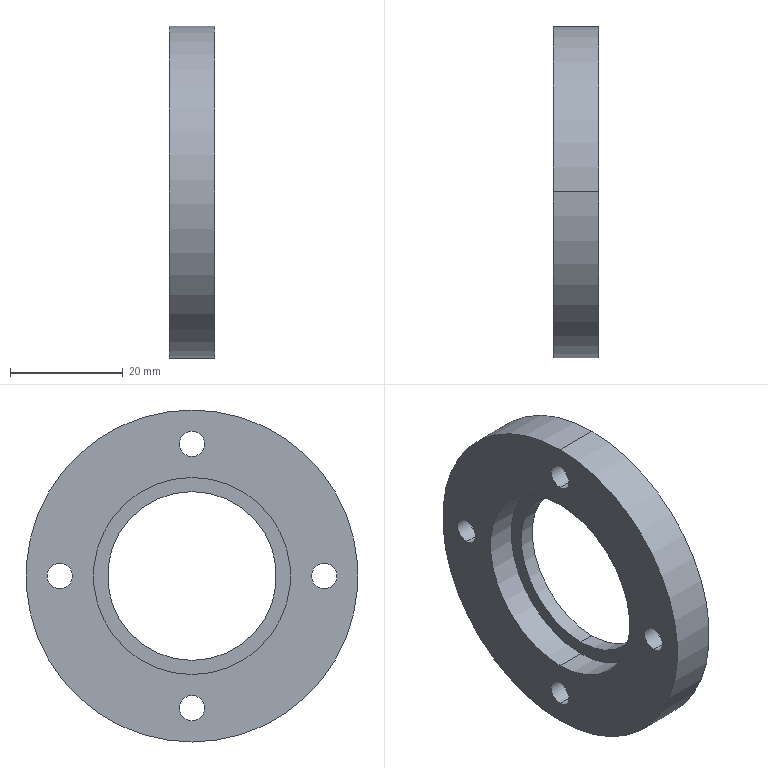Component | SolidWorks | JF21-110.1-33-1-SOLID1-1 | 1 solid | 29 faces | box 8 x 59 x 59 mm | volume 13564 mm3 | cylinder 22 | plane 7 | commonest cylinder face diameters 8.5 x8 4.5 x8 35 x2 59 x2 30 x2
STEP:
#1=COLOUR_RGB('',0.7922,0.8196,0.9333);
#2=FILL_AREA_STYLE_COLOUR('',#1);
#3=FILL_AREA_STYLE('',(#2));
#4=SURFACE_STYLE_FILL_AREA(#3);
#5=SURFACE_SIDE_STYLE('',(#4));
#6=SURFACE_STYLE_USAGE(.BOTH.,#5);
#7=PRESENTATION_STYLE_ASSIGNMENT((#6));
#8=CARTESIAN_POINT('',(17.165,-17.52,23.927));
#9=VERTEX_POINT('',#8);
#10=CARTESIAN_POINT('',(17.165,-17.52,23.593));
#11=VERTEX_POINT('',#10);
#12=CARTESIAN_POINT('',(17.165,-17.52,23.76));
#13=DIRECTION('',(1.,0.,0.));
#14=DIRECTION('',(0.,0.,-1.));
#15=AXIS2_PLACEMENT_3D('',#12,#13,#14);
#16=CIRCLE('',#15,0.1673);
#17=EDGE_CURVE('',#9,#11,#16,.T.);
#18=ORIENTED_EDGE('',*,*,#17,.F.);
#19=CARTESIAN_POINT('',(17.362,-17.52,23.927));
#20=VERTEX_POINT('',#19);
#21=CARTESIAN_POINT('',(17.362,-17.52,23.927));
#22=DIRECTION('',(-1.,0.,0.));
#23=VECTOR('',#22,39.37);
#24=LINE('',#21,#23);
#25=EDGE_CURVE('',#20,#9,#24,.T.);
#26=ORIENTED_EDGE('',*,*,#25,.F.);
#27=CARTESIAN_POINT('',(17.362,-17.52,23.593));
#28=VERTEX_POINT('',#27);
#29=CARTESIAN_POINT('',(17.362,-17.52,23.76));
#30=DIRECTION('',(1.,0.,0.));
#31=DIRECTION('',(0.,0.,-1.));
#32=AXIS2_PLACEMENT_3D('',#29,#30,#31);
#33=CIRCLE('',#32,0.1673);
#34=EDGE_CURVE('',#20,#28,#33,.T.);
#35=ORIENTED_EDGE('',*,*,#34,.T.);
#36=CARTESIAN_POINT('',(17.362,-17.52,23.593));
#37=DIRECTION('',(-1.,0.,0.));
#38=VECTOR('',#37,39.37);
#39=LINE('',#36,#38);
#40=EDGE_CURVE('',#28,#11,#39,.T.);
#41=ORIENTED_EDGE('',*,*,#40,.T.);
#42=EDGE_LOOP('',(#18,#26,#35,#41));
#43=FACE_OUTER_BOUND('',#42,.T.);
#44=CARTESIAN_POINT('',(17.362,-17.52,23.76));
#45=DIRECTION('',(1.,0.,0.));
#46=DIRECTION('',(0.,0.,1.));
#47=AXIS2_PLACEMENT_3D('',#44,#45,#46);
#48=CYLINDRICAL_SURFACE('',#47,0.1673);
#49=ADVANCED_FACE('',(#43),#48,.F.);
#50=CARTESIAN_POINT('',(17.047,-17.52,23.848));
#51=VERTEX_POINT('',#50);
#52=CARTESIAN_POINT('',(17.047,-17.52,23.671));
#53=VERTEX_POINT('',#52);
#54=CARTESIAN_POINT('',(17.047,-17.52,23.76));
#55=DIRECTION('',(1.,0.,0.));
#56=DIRECTION('',(0.,0.,-1.));
#57=AXIS2_PLACEMENT_3D('',#54,#55,#56);
#58=CIRCLE('',#57,0.08858);
#59=EDGE_CURVE('',#51,#53,#58,.T.);
#60=ORIENTED_EDGE('',*,*,#59,.F.);
#61=CARTESIAN_POINT('',(17.165,-17.52,23.848));
#62=VERTEX_POINT('',#61);
#63=CARTESIAN_POINT('',(17.362,-17.52,23.848));
#64=DIRECTION('',(-1.,0.,0.));
#65=VECTOR('',#64,39.37);
#66=LINE('',#63,#65);
#67=EDGE_CURVE('',#62,#51,#66,.T.);
#68=ORIENTED_EDGE('',*,*,#67,.F.);
#69=CARTESIAN_POINT('',(17.165,-17.52,23.671));
#70=VERTEX_POINT('',#69);
#71=CARTESIAN_POINT('',(17.165,-17.52,23.76));
#72=DIRECTION('',(1.,0.,0.));
#73=DIRECTION('',(0.,0.,-1.));
#74=AXIS2_PLACEMENT_3D('',#71,#72,#73);
#75=CIRCLE('',#74,0.08858);
#76=EDGE_CURVE('',#62,#70,#75,.T.);
#77=ORIENTED_EDGE('',*,*,#76,.T.);
#78=CARTESIAN_POINT('',(17.362,-17.52,23.671));
#79=DIRECTION('',(-1.,0.,0.));
#80=VECTOR('',#79,39.37);
#81=LINE('',#78,#80);
#82=EDGE_CURVE('',#70,#53,#81,.T.);
#83=ORIENTED_EDGE('',*,*,#82,.T.);
#84=EDGE_LOOP('',(#60,#68,#77,#83));
#85=FACE_OUTER_BOUND('',#84,.T.);
#86=CARTESIAN_POINT('',(17.362,-17.52,23.76));
#87=DIRECTION('',(1.,0.,0.));
#88=DIRECTION('',(0.,0.,1.));
#89=AXIS2_PLACEMENT_3D('',#86,#87,#88);
#90=CYLINDRICAL_SURFACE('',#89,0.08858);
#91=ADVANCED_FACE('',(#85),#90,.F.);
#92=CARTESIAN_POINT('',(17.165,-18.445,23.002));
#93=VERTEX_POINT('',#92);
#94=CARTESIAN_POINT('',(17.165,-18.445,22.667));
#95=VERTEX_POINT('',#94);
#96=CARTESIAN_POINT('',(17.165,-18.445,22.835));
#97=DIRECTION('',(1.,0.,0.));
#98=DIRECTION('',(0.,0.,-1.));
#99=AXIS2_PLACEMENT_3D('',#96,#97,#98);
#100=CIRCLE('',#99,0.1673);
#101=EDGE_CURVE('',#93,#95,#100,.T.);
#102=ORIENTED_EDGE('',*,*,#101,.F.);
#103=CARTESIAN_POINT('',(17.362,-18.445,23.002));
#104=VERTEX_POINT('',#103);
#105=CARTESIAN_POINT('',(17.362,-18.445,23.002));
#106=DIRECTION('',(-1.,0.,0.));
#107=VECTOR('',#106,39.37);
#108=LINE('',#105,#107);
#109=EDGE_CURVE('',#104,#93,#108,.T.);
#110=ORIENTED_EDGE('',*,*,#109,.F.);
#111=CARTESIAN_POINT('',(17.362,-18.445,22.667));
#112=VERTEX_POINT('',#111);
#113=CARTESIAN_POINT('',(17.362,-18.445,22.835));
#114=DIRECTION('',(1.,0.,0.));
#115=DIRECTION('',(0.,0.,-1.));
#116=AXIS2_PLACEMENT_3D('',#113,#114,#115);
#117=CIRCLE('',#116,0.1673);
#118=EDGE_CURVE('',#104,#112,#117,.T.);
#119=ORIENTED_EDGE('',*,*,#118,.T.);
#120=CARTESIAN_POINT('',(17.362,-18.445,22.667));
#121=DIRECTION('',(-1.,0.,0.));
#122=VECTOR('',#121,39.37);
#123=LINE('',#120,#122);
#124=EDGE_CURVE('',#112,#95,#123,.T.);
#125=ORIENTED_EDGE('',*,*,#124,.T.);
#126=EDGE_LOOP('',(#102,#110,#119,#125));
#127=FACE_OUTER_BOUND('',#126,.T.);
#128=CARTESIAN_POINT('',(17.362,-18.445,22.835));
#129=DIRECTION('',(1.,0.,0.));
#130=DIRECTION('',(0.,0.,1.));
#131=AXIS2_PLACEMENT_3D('',#128,#129,#130);
#132=CYLINDRICAL_SURFACE('',#131,0.1673);
#133=ADVANCED_FACE('',(#127),#132,.F.);
#134=CARTESIAN_POINT('',(17.047,-18.445,22.923));
#135=VERTEX_POINT('',#134);
#136=CARTESIAN_POINT('',(17.047,-18.445,22.746));
#137=VERTEX_POINT('',#136);
#138=CARTESIAN_POINT('',(17.047,-18.445,22.835));
#139=DIRECTION('',(1.,0.,0.));
#140=DIRECTION('',(0.,0.,-1.));
#141=AXIS2_PLACEMENT_3D('',#138,#139,#140);
#142=CIRCLE('',#141,0.08858);
#143=EDGE_CURVE('',#135,#137,#142,.T.);
#144=ORIENTED_EDGE('',*,*,#143,.F.);
#145=CARTESIAN_POINT('',(17.165,-18.445,22.923));
#146=VERTEX_POINT('',#145);
#147=CARTESIAN_POINT('',(17.362,-18.445,22.923));
#148=DIRECTION('',(-1.,0.,0.));
#149=VECTOR('',#148,39.37);
#150=LINE('',#147,#149);
#151=EDGE_CURVE('',#146,#135,#150,.T.);
#152=ORIENTED_EDGE('',*,*,#151,.F.);
#153=CARTESIAN_POINT('',(17.165,-18.445,22.746));
#154=VERTEX_POINT('',#153);
#155=CARTESIAN_POINT('',(17.165,-18.445,22.835));
#156=DIRECTION('',(1.,0.,0.));
#157=DIRECTION('',(0.,0.,-1.));
#158=AXIS2_PLACEMENT_3D('',#155,#156,#157);
#159=CIRCLE('',#158,0.08858);
#160=EDGE_CURVE('',#146,#154,#159,.T.);
#161=ORIENTED_EDGE('',*,*,#160,.T.);
#162=CARTESIAN_POINT('',(17.362,-18.445,22.746));
#163=DIRECTION('',(-1.,0.,0.));
#164=VECTOR('',#163,39.37);
#165=LINE('',#162,#164);
#166=EDGE_CURVE('',#154,#137,#165,.T.);
#167=ORIENTED_EDGE('',*,*,#166,.T.);
#168=EDGE_LOOP('',(#144,#152,#161,#167));
#169=FACE_OUTER_BOUND('',#168,.T.);
#170=CARTESIAN_POINT('',(17.362,-18.445,22.835));
#171=DIRECTION('',(1.,0.,0.));
#172=DIRECTION('',(0.,0.,1.));
#173=AXIS2_PLACEMENT_3D('',#170,#171,#172);
#174=CYLINDRICAL_SURFACE('',#173,0.08858);
#175=ADVANCED_FACE('',(#169),#174,.F.);
#176=CARTESIAN_POINT('',(17.165,-17.52,22.077));
#177=VERTEX_POINT('',#176);
#178=CARTESIAN_POINT('',(17.165,-17.52,21.742));
#179=VERTEX_POINT('',#178);
#180=CARTESIAN_POINT('',(17.165,-17.52,21.909));
#181=DIRECTION('',(1.,0.,0.));
#182=DIRECTION('',(0.,0.,-1.));
#183=AXIS2_PLACEMENT_3D('',#180,#181,#182);
#184=CIRCLE('',#183,0.1673);
#185=EDGE_CURVE('',#177,#179,#184,.T.);
#186=ORIENTED_EDGE('',*,*,#185,.F.);
#187=CARTESIAN_POINT('',(17.362,-17.52,22.077));
#188=VERTEX_POINT('',#187);
#189=CARTESIAN_POINT('',(17.362,-17.52,22.077));
#190=DIRECTION('',(-1.,0.,0.));
#191=VECTOR('',#190,39.37);
#192=LINE('',#189,#191);
#193=EDGE_CURVE('',#188,#177,#192,.T.);
#194=ORIENTED_EDGE('',*,*,#193,.F.);
#195=CARTESIAN_POINT('',(17.362,-17.52,21.742));
#196=VERTEX_POINT('',#195);
#197=CARTESIAN_POINT('',(17.362,-17.52,21.909));
#198=DIRECTION('',(1.,0.,0.));
#199=DIRECTION('',(0.,0.,-1.));
#200=AXIS2_PLACEMENT_3D('',#197,#198,#199);
#201=CIRCLE('',#200,0.1673);
#202=EDGE_CURVE('',#188,#196,#201,.T.);
#203=ORIENTED_EDGE('',*,*,#202,.T.);
#204=CARTESIAN_POINT('',(17.362,-17.52,21.742));
#205=DIRECTION('',(-1.,0.,0.));
#206=VECTOR('',#205,39.37);
#207=LINE('',#204,#206);
#208=EDGE_CURVE('',#196,#179,#207,.T.);
#209=ORIENTED_EDGE('',*,*,#208,.T.);
#210=EDGE_LOOP('',(#186,#194,#203,#209));
#211=FACE_OUTER_BOUND('',#210,.T.);
#212=CARTESIAN_POINT('',(17.362,-17.52,21.909));
#213=DIRECTION('',(1.,0.,0.));
#214=DIRECTION('',(0.,0.,1.));
#215=AXIS2_PLACEMENT_3D('',#212,#213,#214);
#216=CYLINDRICAL_SURFACE('',#215,0.1673);
#217=ADVANCED_FACE('',(#211),#216,.F.);
#218=CARTESIAN_POINT('',(17.047,-17.52,21.998));
#219=VERTEX_POINT('',#218);
#220=CARTESIAN_POINT('',(17.047,-17.52,21.821));
#221=VERTEX_POINT('',#220);
#222=CARTESIAN_POINT('',(17.047,-17.52,21.909));
#223=DIRECTION('',(1.,0.,0.));
#224=DIRECTION('',(0.,0.,-1.));
#225=AXIS2_PLACEMENT_3D('',#222,#223,#224);
#226=CIRCLE('',#225,0.08858);
#227=EDGE_CURVE('',#219,#221,#226,.T.);
#228=ORIENTED_EDGE('',*,*,#227,.F.);
#229=CARTESIAN_POINT('',(17.165,-17.52,21.998));
#230=VERTEX_POINT('',#229);
#231=CARTESIAN_POINT('',(17.362,-17.52,21.998));
#232=DIRECTION('',(-1.,0.,0.));
#233=VECTOR('',#232,39.37);
#234=LINE('',#231,#233);
#235=EDGE_CURVE('',#230,#219,#234,.T.);
#236=ORIENTED_EDGE('',*,*,#235,.F.);
#237=CARTESIAN_POINT('',(17.165,-17.52,21.821));
#238=VERTEX_POINT('',#237);
#239=CARTESIAN_POINT('',(17.165,-17.52,21.909));
#240=DIRECTION('',(1.,0.,0.));
#241=DIRECTION('',(0.,0.,-1.));
#242=AXIS2_PLACEMENT_3D('',#239,#240,#241);
#243=CIRCLE('',#242,0.08858);
#244=EDGE_CURVE('',#230,#238,#243,.T.);
#245=ORIENTED_EDGE('',*,*,#244,.T.);
#246=CARTESIAN_POINT('',(17.362,-17.52,21.821));
#247=DIRECTION('',(-1.,0.,0.));
#248=VECTOR('',#247,39.37);
#249=LINE('',#246,#248);
#250=EDGE_CURVE('',#238,#221,#249,.T.);
#251=ORIENTED_EDGE('',*,*,#250,.T.);
#252=EDGE_LOOP('',(#228,#236,#245,#251));
#253=FACE_OUTER_BOUND('',#252,.T.);
#254=CARTESIAN_POINT('',(17.362,-17.52,21.909));
#255=DIRECTION('',(1.,0.,0.));
#256=DIRECTION('',(0.,0.,1.));
#257=AXIS2_PLACEMENT_3D('',#254,#255,#256);
#258=CYLINDRICAL_SURFACE('',#257,0.08858);
#259=ADVANCED_FACE('',(#253),#258,.F.);
#260=CARTESIAN_POINT('',(17.165,-16.594,23.002));
#261=VERTEX_POINT('',#260);
#262=CARTESIAN_POINT('',(17.165,-16.594,22.667));
#263=VERTEX_POINT('',#262);
#264=CARTESIAN_POINT('',(17.165,-16.594,22.835));
#265=DIRECTION('',(1.,0.,0.));
#266=DIRECTION('',(0.,0.,-1.));
#267=AXIS2_PLACEMENT_3D('',#264,#265,#266);
#268=CIRCLE('',#267,0.1673);
#269=EDGE_CURVE('',#261,#263,#268,.T.);
#270=ORIENTED_EDGE('',*,*,#269,.F.);
#271=CARTESIAN_POINT('',(17.362,-16.594,23.002));
#272=VERTEX_POINT('',#271);
#273=CARTESIAN_POINT('',(17.362,-16.594,23.002));
#274=DIRECTION('',(-1.,0.,0.));
#275=VECTOR('',#274,39.37);
#276=LINE('',#273,#275);
#277=EDGE_CURVE('',#272,#261,#276,.T.);
#278=ORIENTED_EDGE('',*,*,#277,.F.);
#279=CARTESIAN_POINT('',(17.362,-16.594,22.667));
#280=VERTEX_POINT('',#279);
#281=CARTESIAN_POINT('',(17.362,-16.594,22.835));
#282=DIRECTION('',(1.,0.,0.));
#283=DIRECTION('',(0.,0.,-1.));
#284=AXIS2_PLACEMENT_3D('',#281,#282,#283);
#285=CIRCLE('',#284,0.1673);
#286=EDGE_CURVE('',#272,#280,#285,.T.);
#287=ORIENTED_EDGE('',*,*,#286,.T.);
#288=CARTESIAN_POINT('',(17.362,-16.594,22.667));
#289=DIRECTION('',(-1.,0.,0.));
#290=VECTOR('',#289,39.37);
#291=LINE('',#288,#290);
#292=EDGE_CURVE('',#280,#263,#291,.T.);
#293=ORIENTED_EDGE('',*,*,#292,.T.);
#294=EDGE_LOOP('',(#270,#278,#287,#293));
#295=FACE_OUTER_BOUND('',#294,.T.);
#296=CARTESIAN_POINT('',(17.362,-16.594,22.835));
#297=DIRECTION('',(1.,0.,0.));
#298=DIRECTION('',(0.,0.,1.));
#299=AXIS2_PLACEMENT_3D('',#296,#297,#298);
#300=CYLINDRICAL_SURFACE('',#299,0.1673);
#301=ADVANCED_FACE('',(#295),#300,.F.);
#302=CARTESIAN_POINT('',(17.047,-16.594,22.923));
#303=VERTEX_POINT('',#302);
#304=CARTESIAN_POINT('',(17.047,-16.594,22.746));
#305=VERTEX_POINT('',#304);
#306=CARTESIAN_POINT('',(17.047,-16.594,22.835));
#307=DIRECTION('',(1.,0.,0.));
#308=DIRECTION('',(0.,0.,-1.));
#309=AXIS2_PLACEMENT_3D('',#306,#307,#308);
#310=CIRCLE('',#309,0.08858);
#311=EDGE_CURVE('',#303,#305,#310,.T.);
#312=ORIENTED_EDGE('',*,*,#311,.F.);
#313=CARTESIAN_POINT('',(17.165,-16.594,22.923));
#314=VERTEX_POINT('',#313);
#315=CARTESIAN_POINT('',(17.362,-16.594,22.923));
#316=DIRECTION('',(-1.,0.,0.));
#317=VECTOR('',#316,39.37);
#318=LINE('',#315,#317);
#319=EDGE_CURVE('',#314,#303,#318,.T.);
#320=ORIENTED_EDGE('',*,*,#319,.F.);
#321=CARTESIAN_POINT('',(17.165,-16.594,22.746));
#322=VERTEX_POINT('',#321);
#323=CARTESIAN_POINT('',(17.165,-16.594,22.835));
#324=DIRECTION('',(1.,0.,0.));
#325=DIRECTION('',(0.,0.,-1.));
#326=AXIS2_PLACEMENT_3D('',#323,#324,#325);
#327=CIRCLE('',#326,0.08858);
#328=EDGE_CURVE('',#314,#322,#327,.T.);
#329=ORIENTED_EDGE('',*,*,#328,.T.);
#330=CARTESIAN_POINT('',(17.362,-16.594,22.746));
#331=DIRECTION('',(-1.,0.,0.));
#332=VECTOR('',#331,39.37);
#333=LINE('',#330,#332);
#334=EDGE_CURVE('',#322,#305,#333,.T.);
#335=ORIENTED_EDGE('',*,*,#334,.T.);
#336=EDGE_LOOP('',(#312,#320,#329,#335));
#337=FACE_OUTER_BOUND('',#336,.T.);
#338=CARTESIAN_POINT('',(17.362,-16.594,22.835));
#339=DIRECTION('',(1.,0.,0.));
#340=DIRECTION('',(0.,0.,1.));
#341=AXIS2_PLACEMENT_3D('',#338,#339,#340);
#342=CYLINDRICAL_SURFACE('',#341,0.08858);
#343=ADVANCED_FACE('',(#337),#342,.F.);
#344=CARTESIAN_POINT('',(17.252,-17.52,22.146));
#345=VERTEX_POINT('',#344);
#346=CARTESIAN_POINT('',(17.252,-17.52,23.524));
#347=VERTEX_POINT('',#346);
#348=CARTESIAN_POINT('',(17.252,-17.52,22.835));
#349=DIRECTION('',(-1.,0.,0.));
#350=DIRECTION('',(0.,0.,1.));
#351=AXIS2_PLACEMENT_3D('',#348,#349,#350);
#352=CIRCLE('',#351,0.689);
#353=EDGE_CURVE('',#345,#347,#352,.T.);
#354=ORIENTED_EDGE('',*,*,#353,.F.);
#355=CARTESIAN_POINT('',(17.047,-17.52,22.146));
#356=VERTEX_POINT('',#355);
#357=CARTESIAN_POINT('',(17.252,-17.52,22.146));
#358=DIRECTION('',(-1.,0.,0.));
#359=VECTOR('',#358,39.37);
#360=LINE('',#357,#359);
#361=EDGE_CURVE('',#345,#356,#360,.T.);
#362=ORIENTED_EDGE('',*,*,#361,.T.);
#363=CARTESIAN_POINT('',(17.047,-17.52,23.524));
#364=VERTEX_POINT('',#363);
#365=CARTESIAN_POINT('',(17.047,-17.52,22.835));
#366=DIRECTION('',(-1.,0.,0.));
#367=DIRECTION('',(0.,0.,1.));
#368=AXIS2_PLACEMENT_3D('',#365,#366,#367);
#369=CIRCLE('',#368,0.689);
#370=EDGE_CURVE('',#356,#364,#369,.T.);
#371=ORIENTED_EDGE('',*,*,#370,.T.);
#372=CARTESIAN_POINT('',(17.252,-17.52,23.524));
#373=DIRECTION('',(-1.,0.,0.));
#374=VECTOR('',#373,39.37);
#375=LINE('',#372,#374);
#376=EDGE_CURVE('',#347,#364,#375,.T.);
#377=ORIENTED_EDGE('',*,*,#376,.F.);
#378=EDGE_LOOP('',(#354,#362,#371,#377));
#379=FACE_OUTER_BOUND('',#378,.T.);
#380=CARTESIAN_POINT('',(17.252,-17.52,22.835));
#381=DIRECTION('',(-1.,0.,0.));
#382=DIRECTION('',(0.,0.,-1.));
#383=AXIS2_PLACEMENT_3D('',#380,#381,#382);
#384=CYLINDRICAL_SURFACE('',#383,0.689);
#385=ADVANCED_FACE('',(#379),#384,.F.);
#386=CARTESIAN_POINT('',(17.362,-17.52,21.673));
#387=VERTEX_POINT('',#386);
#388=CARTESIAN_POINT('',(17.362,-17.52,23.996));
#389=VERTEX_POINT('',#388);
#390=CARTESIAN_POINT('',(17.362,-17.52,22.835));
#391=DIRECTION('',(1.,0.,0.));
#392=DIRECTION('',(0.,0.,-1.));
#393=AXIS2_PLACEMENT_3D('',#390,#391,#392);
#394=CIRCLE('',#393,1.161);
#395=EDGE_CURVE('',#387,#389,#394,.T.);
#396=ORIENTED_EDGE('',*,*,#395,.F.);
#397=CARTESIAN_POINT('',(17.047,-17.52,21.673));
#398=VERTEX_POINT('',#397);
#399=CARTESIAN_POINT('',(17.362,-17.52,21.673));
#400=DIRECTION('',(-1.,0.,0.));
#401=VECTOR('',#400,39.37);
#402=LINE('',#399,#401);
#403=EDGE_CURVE('',#387,#398,#402,.T.);
#404=ORIENTED_EDGE('',*,*,#403,.T.);
#405=CARTESIAN_POINT('',(17.047,-17.52,23.996));
#406=VERTEX_POINT('',#405);
#407=CARTESIAN_POINT('',(17.047,-17.52,22.835));
#408=DIRECTION('',(1.,0.,0.));
#409=DIRECTION('',(0.,0.,-1.));
#410=AXIS2_PLACEMENT_3D('',#407,#408,#409);
#411=CIRCLE('',#410,1.161);
#412=EDGE_CURVE('',#398,#406,#411,.T.);
#413=ORIENTED_EDGE('',*,*,#412,.T.);
#414=CARTESIAN_POINT('',(17.362,-17.52,23.996));
#415=DIRECTION('',(-1.,0.,0.));
#416=VECTOR('',#415,39.37);
#417=LINE('',#414,#416);
#418=EDGE_CURVE('',#389,#406,#417,.T.);
#419=ORIENTED_EDGE('',*,*,#418,.F.);
#420=EDGE_LOOP('',(#396,#404,#413,#419));
#421=FACE_OUTER_BOUND('',#420,.T.);
#422=CARTESIAN_POINT('',(17.362,-17.52,22.835));
#423=DIRECTION('',(-1.,0.,0.));
#424=DIRECTION('',(0.,0.,-1.));
#425=AXIS2_PLACEMENT_3D('',#422,#423,#424);
#426=CYLINDRICAL_SURFACE('',#425,1.161);
#427=ADVANCED_FACE('',(#421),#426,.T.);
#428=CARTESIAN_POINT('',(17.362,-17.52,22.244));
#429=VERTEX_POINT('',#428);
#430=CARTESIAN_POINT('',(17.362,-17.52,23.425));
#431=VERTEX_POINT('',#430);
#432=CARTESIAN_POINT('',(17.362,-17.52,22.835));
#433=DIRECTION('',(-1.,0.,0.));
#434=DIRECTION('',(0.,0.,1.));
#435=AXIS2_PLACEMENT_3D('',#432,#433,#434);
#436=CIRCLE('',#435,0.5906);
#437=EDGE_CURVE('',#429,#431,#436,.T.);
#438=ORIENTED_EDGE('',*,*,#437,.F.);
#439=CARTESIAN_POINT('',(17.252,-17.52,22.244));
#440=VERTEX_POINT('',#439);
#441=CARTESIAN_POINT('',(17.362,-17.52,22.244));
#442=DIRECTION('',(-1.,0.,0.));
#443=VECTOR('',#442,39.37);
#444=LINE('',#441,#443);
#445=EDGE_CURVE('',#429,#440,#444,.T.);
#446=ORIENTED_EDGE('',*,*,#445,.T.);
#447=CARTESIAN_POINT('',(17.252,-17.52,23.425));
#448=VERTEX_POINT('',#447);
#449=CARTESIAN_POINT('',(17.252,-17.52,22.835));
#450=DIRECTION('',(1.,0.,0.));
#451=DIRECTION('',(0.,0.,1.));
#452=AXIS2_PLACEMENT_3D('',#449,#450,#451);
#453=CIRCLE('',#452,0.5906);
#454=EDGE_CURVE('',#448,#440,#453,.T.);
#455=ORIENTED_EDGE('',*,*,#454,.F.);
#456=CARTESIAN_POINT('',(17.362,-17.52,23.425));
#457=DIRECTION('',(-1.,0.,0.));
#458=VECTOR('',#457,39.37);
#459=LINE('',#456,#458);
#460=EDGE_CURVE('',#431,#448,#459,.T.);
#461=ORIENTED_EDGE('',*,*,#460,.F.);
#462=EDGE_LOOP('',(#438,#446,#455,#461));
#463=FACE_OUTER_BOUND('',#462,.T.);
#464=CARTESIAN_POINT('',(17.362,-17.52,22.835));
#465=DIRECTION('',(-1.,0.,0.));
#466=DIRECTION('',(0.,0.,-1.));
#467=AXIS2_PLACEMENT_3D('',#464,#465,#466);
#468=CYLINDRICAL_SURFACE('',#467,0.5906);
#469=ADVANCED_FACE('',(#463),#468,.F.);
#470=ORIENTED_EDGE('',*,*,#445,.F.);
#471=CARTESIAN_POINT('',(17.362,-17.52,22.835));
#472=DIRECTION('',(-1.,0.,0.));
#473=DIRECTION('',(0.,0.,1.));
#474=AXIS2_PLACEMENT_3D('',#471,#472,#473);
#475=CIRCLE('',#474,0.5906);
#476=EDGE_CURVE('',#431,#429,#475,.T.);
#477=ORIENTED_EDGE('',*,*,#476,.F.);
#478=ORIENTED_EDGE('',*,*,#460,.T.);
#479=CARTESIAN_POINT('',(17.252,-17.52,22.835));
#480=DIRECTION('',(1.,0.,0.));
#481=DIRECTION('',(0.,0.,1.));
#482=AXIS2_PLACEMENT_3D('',#479,#480,#481);
#483=CIRCLE('',#482,0.5906);
#484=EDGE_CURVE('',#440,#448,#483,.T.);
#485=ORIENTED_EDGE('',*,*,#484,.F.);
#486=EDGE_LOOP('',(#470,#477,#478,#485));
#487=FACE_OUTER_BOUND('',#486,.T.);
#488=CARTESIAN_POINT('',(17.362,-17.52,22.835));
#489=DIRECTION('',(-1.,0.,0.));
#490=DIRECTION('',(0.,0.,-1.));
#491=AXIS2_PLACEMENT_3D('',#488,#489,#490);
#492=CYLINDRICAL_SURFACE('',#491,0.5906);
#493=ADVANCED_FACE('',(#487),#492,.F.);
#494=ORIENTED_EDGE('',*,*,#403,.F.);
#495=CARTESIAN_POINT('',(17.362,-17.52,22.835));
#496=DIRECTION('',(1.,0.,0.));
#497=DIRECTION('',(0.,0.,-1.));
#498=AXIS2_PLACEMENT_3D('',#495,#496,#497);
#499=CIRCLE('',#498,1.161);
#500=EDGE_CURVE('',#389,#387,#499,.T.);
#501=ORIENTED_EDGE('',*,*,#500,.F.);
#502=ORIENTED_EDGE('',*,*,#418,.T.);
#503=CARTESIAN_POINT('',(17.047,-17.52,22.835));
#504=DIRECTION('',(1.,0.,0.));
#505=DIRECTION('',(0.,0.,-1.));
#506=AXIS2_PLACEMENT_3D('',#503,#504,#505);
#507=CIRCLE('',#506,1.161);
#508=EDGE_CURVE('',#406,#398,#507,.T.);
#509=ORIENTED_EDGE('',*,*,#508,.T.);
#510=EDGE_LOOP('',(#494,#501,#502,#509));
#511=FACE_OUTER_BOUND('',#510,.T.);
#512=CARTESIAN_POINT('',(17.362,-17.52,22.835));
#513=DIRECTION('',(-1.,0.,0.));
#514=DIRECTION('',(0.,0.,-1.));
#515=AXIS2_PLACEMENT_3D('',#512,#513,#514);
#516=CYLINDRICAL_SURFACE('',#515,1.161);
#517=ADVANCED_FACE('',(#511),#516,.T.);
#518=CARTESIAN_POINT('',(17.362,-17.52,23.76));
#519=DIRECTION('',(1.,0.,0.));
#520=DIRECTION('',(0.,0.,-1.));
#521=AXIS2_PLACEMENT_3D('',#518,#519,#520);
#522=CIRCLE('',#521,0.1673);
#523=EDGE_CURVE('',#28,#20,#522,.T.);
#524=ORIENTED_EDGE('',*,*,#523,.F.);
#525=ORIENTED_EDGE('',*,*,#34,.F.);
#526=EDGE_LOOP('',(#524,#525));
#527=FACE_BOUND('',#526,.T.);
#528=CARTESIAN_POINT('',(17.362,-18.445,22.835));
#529=DIRECTION('',(1.,0.,0.));
#530=DIRECTION('',(0.,0.,-1.));
#531=AXIS2_PLACEMENT_3D('',#528,#529,#530);
#532=CIRCLE('',#531,0.1673);
#533=EDGE_CURVE('',#112,#104,#532,.T.);
#534=ORIENTED_EDGE('',*,*,#533,.F.);
#535=ORIENTED_EDGE('',*,*,#118,.F.);
#536=EDGE_LOOP('',(#534,#535));
#537=FACE_BOUND('',#536,.T.);
#538=CARTESIAN_POINT('',(17.362,-17.52,21.909));
#539=DIRECTION('',(1.,0.,0.));
#540=DIRECTION('',(0.,0.,-1.));
#541=AXIS2_PLACEMENT_3D('',#538,#539,#540);
#542=CIRCLE('',#541,0.1673);
#543=EDGE_CURVE('',#196,#188,#542,.T.);
#544=ORIENTED_EDGE('',*,*,#543,.F.);
#545=ORIENTED_EDGE('',*,*,#202,.F.);
#546=EDGE_LOOP('',(#544,#545));
#547=FACE_BOUND('',#546,.T.);
#548=CARTESIAN_POINT('',(17.362,-16.594,22.835));
#549=DIRECTION('',(1.,0.,0.));
#550=DIRECTION('',(0.,0.,-1.));
#551=AXIS2_PLACEMENT_3D('',#548,#549,#550);
#552=CIRCLE('',#551,0.1673);
#553=EDGE_CURVE('',#280,#272,#552,.T.);
#554=ORIENTED_EDGE('',*,*,#553,.F.);
#555=ORIENTED_EDGE('',*,*,#286,.F.);
#556=EDGE_LOOP('',(#554,#555));
#557=FACE_BOUND('',#556,.T.);
#558=ORIENTED_EDGE('',*,*,#476,.T.);
#559=ORIENTED_EDGE('',*,*,#437,.T.);
#560=EDGE_LOOP('',(#558,#559));
#561=FACE_BOUND('',#560,.T.);
#562=ORIENTED_EDGE('',*,*,#500,.T.);
#563=ORIENTED_EDGE('',*,*,#395,.T.);
#564=EDGE_LOOP('',(#562,#563));
#565=FACE_OUTER_BOUND('',#564,.T.);
#566=CARTESIAN_POINT('',(17.362,-17.52,22.835));
#567=DIRECTION('',(1.,0.,0.));
#568=DIRECTION('',(0.,0.,1.));
#569=AXIS2_PLACEMENT_3D('',#566,#567,#568);
#570=PLANE('',#569);
#571=ADVANCED_FACE('',(#527,#537,#547,#557,#561,#565),#570,.T.);
#572=CARTESIAN_POINT('',(17.047,-17.52,23.76));
#573=DIRECTION('',(1.,0.,0.));
#574=DIRECTION('',(0.,0.,-1.));
#575=AXIS2_PLACEMENT_3D('',#572,#573,#574);
#576=CIRCLE('',#575,0.08858);
#577=EDGE_CURVE('',#53,#51,#576,.T.);
#578=ORIENTED_EDGE('',*,*,#577,.T.);
#579=ORIENTED_EDGE('',*,*,#59,.T.);
#580=EDGE_LOOP('',(#578,#579));
#581=FACE_BOUND('',#580,.T.);
#582=CARTESIAN_POINT('',(17.047,-18.445,22.835));
#583=DIRECTION('',(1.,0.,0.));
#584=DIRECTION('',(0.,0.,-1.));
#585=AXIS2_PLACEMENT_3D('',#582,#583,#584);
#586=CIRCLE('',#585,0.08858);
#587=EDGE_CURVE('',#137,#135,#586,.T.);
#588=ORIENTED_EDGE('',*,*,#587,.T.);
#589=ORIENTED_EDGE('',*,*,#143,.T.);
#590=EDGE_LOOP('',(#588,#589));
#591=FACE_BOUND('',#590,.T.);
#592=CARTESIAN_POINT('',(17.047,-17.52,21.909));
#593=DIRECTION('',(1.,0.,0.));
#594=DIRECTION('',(0.,0.,-1.));
#595=AXIS2_PLACEMENT_3D('',#592,#593,#594);
#596=CIRCLE('',#595,0.08858);
#597=EDGE_CURVE('',#221,#219,#596,.T.);
#598=ORIENTED_EDGE('',*,*,#597,.T.);
#599=ORIENTED_EDGE('',*,*,#227,.T.);
#600=EDGE_LOOP('',(#598,#599));
#601=FACE_BOUND('',#600,.T.);
#602=CARTESIAN_POINT('',(17.047,-16.594,22.835));
#603=DIRECTION('',(1.,0.,0.));
#604=DIRECTION('',(0.,0.,-1.));
#605=AXIS2_PLACEMENT_3D('',#602,#603,#604);
#606=CIRCLE('',#605,0.08858);
#607=EDGE_CURVE('',#305,#303,#606,.T.);
#608=ORIENTED_EDGE('',*,*,#607,.T.);
#609=ORIENTED_EDGE('',*,*,#311,.T.);
#610=EDGE_LOOP('',(#608,#609));
#611=FACE_BOUND('',#610,.T.);
#612=CARTESIAN_POINT('',(17.047,-17.52,22.835));
#613=DIRECTION('',(-1.,0.,0.));
#614=DIRECTION('',(0.,0.,1.));
#615=AXIS2_PLACEMENT_3D('',#612,#613,#614);
#616=CIRCLE('',#615,0.689);
#617=EDGE_CURVE('',#364,#356,#616,.T.);
#618=ORIENTED_EDGE('',*,*,#617,.F.);
#619=ORIENTED_EDGE('',*,*,#370,.F.);
#620=EDGE_LOOP('',(#618,#619));
#621=FACE_BOUND('',#620,.T.);
#622=ORIENTED_EDGE('',*,*,#508,.F.);
#623=ORIENTED_EDGE('',*,*,#412,.F.);
#624=EDGE_LOOP('',(#622,#623));
#625=FACE_OUTER_BOUND('',#624,.T.);
#626=CARTESIAN_POINT('',(17.047,-17.52,22.835));
#627=DIRECTION('',(1.,0.,0.));
#628=DIRECTION('',(0.,0.,1.));
#629=AXIS2_PLACEMENT_3D('',#626,#627,#628);
#630=PLANE('',#629);
#631=ADVANCED_FACE('',(#581,#591,#601,#611,#621,#625),#630,.F.);
#632=CARTESIAN_POINT('',(17.252,-17.52,22.835));
#633=DIRECTION('',(-1.,0.,0.));
#634=DIRECTION('',(0.,0.,1.));
#635=AXIS2_PLACEMENT_3D('',#632,#633,#634);
#636=CIRCLE('',#635,0.689);
#637=EDGE_CURVE('',#347,#345,#636,.T.);
#638=ORIENTED_EDGE('',*,*,#637,.T.);
#639=ORIENTED_EDGE('',*,*,#353,.T.);
#640=EDGE_LOOP('',(#638,#639));
#641=FACE_OUTER_BOUND('',#640,.T.);
#642=ORIENTED_EDGE('',*,*,#454,.T.);
#643=ORIENTED_EDGE('',*,*,#484,.T.);
#644=EDGE_LOOP('',(#642,#643));
#645=FACE_BOUND('',#644,.T.);
#646=CARTESIAN_POINT('',(17.252,-17.52,22.835));
#647=DIRECTION('',(-1.,0.,0.));
#648=DIRECTION('',(0.,0.,-1.));
#649=AXIS2_PLACEMENT_3D('',#646,#647,#648);
#650=PLANE('',#649);
#651=ADVANCED_FACE('',(#641,#645),#650,.T.);
#652=ORIENTED_EDGE('',*,*,#361,.F.);
#653=ORIENTED_EDGE('',*,*,#637,.F.);
#654=ORIENTED_EDGE('',*,*,#376,.T.);
#655=ORIENTED_EDGE('',*,*,#617,.T.);
#656=EDGE_LOOP('',(#652,#653,#654,#655));
#657=FACE_OUTER_BOUND('',#656,.T.);
#658=CARTESIAN_POINT('',(17.252,-17.52,22.835));
#659=DIRECTION('',(-1.,0.,0.));
#660=DIRECTION('',(0.,0.,-1.));
#661=AXIS2_PLACEMENT_3D('',#658,#659,#660);
#662=CYLINDRICAL_SURFACE('',#661,0.689);
#663=ADVANCED_FACE('',(#657),#662,.F.);
#664=ORIENTED_EDGE('',*,*,#319,.T.);
#665=ORIENTED_EDGE('',*,*,#607,.F.);
#666=ORIENTED_EDGE('',*,*,#334,.F.);
#667=CARTESIAN_POINT('',(17.165,-16.594,22.835));
#668=DIRECTION('',(1.,0.,0.));
#669=DIRECTION('',(0.,0.,-1.));
#670=AXIS2_PLACEMENT_3D('',#667,#668,#669);
#671=CIRCLE('',#670,0.08858);
#672=EDGE_CURVE('',#322,#314,#671,.T.);
#673=ORIENTED_EDGE('',*,*,#672,.T.);
#674=EDGE_LOOP('',(#664,#665,#666,#673));
#675=FACE_OUTER_BOUND('',#674,.T.);
#676=CARTESIAN_POINT('',(17.362,-16.594,22.835));
#677=DIRECTION('',(1.,0.,0.));
#678=DIRECTION('',(0.,0.,1.));
#679=AXIS2_PLACEMENT_3D('',#676,#677,#678);
#680=CYLINDRICAL_SURFACE('',#679,0.08858);
#681=ADVANCED_FACE('',(#675),#680,.F.);
#682=ORIENTED_EDGE('',*,*,#672,.F.);
#683=ORIENTED_EDGE('',*,*,#328,.F.);
#684=EDGE_LOOP('',(#682,#683));
#685=FACE_BOUND('',#684,.T.);
#686=CARTESIAN_POINT('',(17.165,-16.594,22.835));
#687=DIRECTION('',(1.,0.,0.));
#688=DIRECTION('',(0.,0.,-1.));
#689=AXIS2_PLACEMENT_3D('',#686,#687,#688);
#690=CIRCLE('',#689,0.1673);
#691=EDGE_CURVE('',#263,#261,#690,.T.);
#692=ORIENTED_EDGE('',*,*,#691,.T.);
#693=ORIENTED_EDGE('',*,*,#269,.T.);
#694=EDGE_LOOP('',(#692,#693));
#695=FACE_OUTER_BOUND('',#694,.T.);
#696=CARTESIAN_POINT('',(17.165,-16.506,22.835));
#697=DIRECTION('',(-1.,0.,0.));
#698=DIRECTION('',(0.,0.,-1.));
#699=AXIS2_PLACEMENT_3D('',#696,#697,#698);
#700=PLANE('',#699);
#701=ADVANCED_FACE('',(#685,#695),#700,.F.);
#702=ORIENTED_EDGE('',*,*,#277,.T.);
#703=ORIENTED_EDGE('',*,*,#691,.F.);
#704=ORIENTED_EDGE('',*,*,#292,.F.);
#705=ORIENTED_EDGE('',*,*,#553,.T.);
#706=EDGE_LOOP('',(#702,#703,#704,#705));
#707=FACE_OUTER_BOUND('',#706,.T.);
#708=CARTESIAN_POINT('',(17.362,-16.594,22.835));
#709=DIRECTION('',(1.,0.,0.));
#710=DIRECTION('',(0.,0.,1.));
#711=AXIS2_PLACEMENT_3D('',#708,#709,#710);
#712=CYLINDRICAL_SURFACE('',#711,0.1673);
#713=ADVANCED_FACE('',(#707),#712,.F.);
#714=ORIENTED_EDGE('',*,*,#235,.T.);
#715=ORIENTED_EDGE('',*,*,#597,.F.);
#716=ORIENTED_EDGE('',*,*,#250,.F.);
#717=CARTESIAN_POINT('',(17.165,-17.52,21.909));
#718=DIRECTION('',(1.,0.,0.));
#719=DIRECTION('',(0.,0.,-1.));
#720=AXIS2_PLACEMENT_3D('',#717,#718,#719);
#721=CIRCLE('',#720,0.08858);
#722=EDGE_CURVE('',#238,#230,#721,.T.);
#723=ORIENTED_EDGE('',*,*,#722,.T.);
#724=EDGE_LOOP('',(#714,#715,#716,#723));
#725=FACE_OUTER_BOUND('',#724,.T.);
#726=CARTESIAN_POINT('',(17.362,-17.52,21.909));
#727=DIRECTION('',(1.,0.,0.));
#728=DIRECTION('',(0.,0.,1.));
#729=AXIS2_PLACEMENT_3D('',#726,#727,#728);
#730=CYLINDRICAL_SURFACE('',#729,0.08858);
#731=ADVANCED_FACE('',(#725),#730,.F.);
#732=ORIENTED_EDGE('',*,*,#722,.F.);
#733=ORIENTED_EDGE('',*,*,#244,.F.);
#734=EDGE_LOOP('',(#732,#733));
#735=FACE_BOUND('',#734,.T.);
#736=CARTESIAN_POINT('',(17.165,-17.52,21.909));
#737=DIRECTION('',(1.,0.,0.));
#738=DIRECTION('',(0.,0.,-1.));
#739=AXIS2_PLACEMENT_3D('',#736,#737,#738);
#740=CIRCLE('',#739,0.1673);
#741=EDGE_CURVE('',#179,#177,#740,.T.);
#742=ORIENTED_EDGE('',*,*,#741,.T.);
#743=ORIENTED_EDGE('',*,*,#185,.T.);
#744=EDGE_LOOP('',(#742,#743));
#745=FACE_OUTER_BOUND('',#744,.T.);
#746=CARTESIAN_POINT('',(17.165,-17.431,21.909));
#747=DIRECTION('',(-1.,0.,0.));
#748=DIRECTION('',(0.,0.,-1.));
#749=AXIS2_PLACEMENT_3D('',#746,#747,#748);
#750=PLANE('',#749);
#751=ADVANCED_FACE('',(#735,#745),#750,.F.);
#752=ORIENTED_EDGE('',*,*,#193,.T.);
#753=ORIENTED_EDGE('',*,*,#741,.F.);
#754=ORIENTED_EDGE('',*,*,#208,.F.);
#755=ORIENTED_EDGE('',*,*,#543,.T.);
#756=EDGE_LOOP('',(#752,#753,#754,#755));
#757=FACE_OUTER_BOUND('',#756,.T.);
#758=CARTESIAN_POINT('',(17.362,-17.52,21.909));
#759=DIRECTION('',(1.,0.,0.));
#760=DIRECTION('',(0.,0.,1.));
#761=AXIS2_PLACEMENT_3D('',#758,#759,#760);
#762=CYLINDRICAL_SURFACE('',#761,0.1673);
#763=ADVANCED_FACE('',(#757),#762,.F.);
#764=ORIENTED_EDGE('',*,*,#151,.T.);
#765=ORIENTED_EDGE('',*,*,#587,.F.);
#766=ORIENTED_EDGE('',*,*,#166,.F.);
#767=CARTESIAN_POINT('',(17.165,-18.445,22.835));
#768=DIRECTION('',(1.,0.,0.));
#769=DIRECTION('',(0.,0.,-1.));
#770=AXIS2_PLACEMENT_3D('',#767,#768,#769);
#771=CIRCLE('',#770,0.08858);
#772=EDGE_CURVE('',#154,#146,#771,.T.);
#773=ORIENTED_EDGE('',*,*,#772,.T.);
#774=EDGE_LOOP('',(#764,#765,#766,#773));
#775=FACE_OUTER_BOUND('',#774,.T.);
#776=CARTESIAN_POINT('',(17.362,-18.445,22.835));
#777=DIRECTION('',(1.,0.,0.));
#778=DIRECTION('',(0.,0.,1.));
#779=AXIS2_PLACEMENT_3D('',#776,#777,#778);
#780=CYLINDRICAL_SURFACE('',#779,0.08858);
#781=ADVANCED_FACE('',(#775),#780,.F.);
#782=ORIENTED_EDGE('',*,*,#772,.F.);
#783=ORIENTED_EDGE('',*,*,#160,.F.);
#784=EDGE_LOOP('',(#782,#783));
#785=FACE_BOUND('',#784,.T.);
#786=CARTESIAN_POINT('',(17.165,-18.445,22.835));
#787=DIRECTION('',(1.,0.,0.));
#788=DIRECTION('',(0.,0.,-1.));
#789=AXIS2_PLACEMENT_3D('',#786,#787,#788);
#790=CIRCLE('',#789,0.1673);
#791=EDGE_CURVE('',#95,#93,#790,.T.);
#792=ORIENTED_EDGE('',*,*,#791,.T.);
#793=ORIENTED_EDGE('',*,*,#101,.T.);
#794=EDGE_LOOP('',(#792,#793));
#795=FACE_OUTER_BOUND('',#794,.T.);
#796=CARTESIAN_POINT('',(17.165,-18.356,22.835));
#797=DIRECTION('',(-1.,0.,0.));
#798=DIRECTION('',(0.,0.,-1.));
#799=AXIS2_PLACEMENT_3D('',#796,#797,#798);
#800=PLANE('',#799);
#801=ADVANCED_FACE('',(#785,#795),#800,.F.);
#802=ORIENTED_EDGE('',*,*,#109,.T.);
#803=ORIENTED_EDGE('',*,*,#791,.F.);
#804=ORIENTED_EDGE('',*,*,#124,.F.);
#805=ORIENTED_EDGE('',*,*,#533,.T.);
#806=EDGE_LOOP('',(#802,#803,#804,#805));
#807=FACE_OUTER_BOUND('',#806,.T.);
#808=CARTESIAN_POINT('',(17.362,-18.445,22.835));
#809=DIRECTION('',(1.,0.,0.));
#810=DIRECTION('',(0.,0.,1.));
#811=AXIS2_PLACEMENT_3D('',#808,#809,#810);
#812=CYLINDRICAL_SURFACE('',#811,0.1673);
#813=ADVANCED_FACE('',(#807),#812,.F.);
#814=ORIENTED_EDGE('',*,*,#67,.T.);
#815=ORIENTED_EDGE('',*,*,#577,.F.);
#816=ORIENTED_EDGE('',*,*,#82,.F.);
#817=CARTESIAN_POINT('',(17.165,-17.52,23.76));
#818=DIRECTION('',(1.,0.,0.));
#819=DIRECTION('',(0.,0.,-1.));
#820=AXIS2_PLACEMENT_3D('',#817,#818,#819);
#821=CIRCLE('',#820,0.08858);
#822=EDGE_CURVE('',#70,#62,#821,.T.);
#823=ORIENTED_EDGE('',*,*,#822,.T.);
#824=EDGE_LOOP('',(#814,#815,#816,#823));
#825=FACE_OUTER_BOUND('',#824,.T.);
#826=CARTESIAN_POINT('',(17.362,-17.52,23.76));
#827=DIRECTION('',(1.,0.,0.));
#828=DIRECTION('',(0.,0.,1.));
#829=AXIS2_PLACEMENT_3D('',#826,#827,#828);
#830=CYLINDRICAL_SURFACE('',#829,0.08858);
#831=ADVANCED_FACE('',(#825),#830,.F.);
#832=ORIENTED_EDGE('',*,*,#822,.F.);
#833=ORIENTED_EDGE('',*,*,#76,.F.);
#834=EDGE_LOOP('',(#832,#833));
#835=FACE_BOUND('',#834,.T.);
#836=CARTESIAN_POINT('',(17.165,-17.52,23.76));
#837=DIRECTION('',(1.,0.,0.));
#838=DIRECTION('',(0.,0.,-1.));
#839=AXIS2_PLACEMENT_3D('',#836,#837,#838);
#840=CIRCLE('',#839,0.1673);
#841=EDGE_CURVE('',#11,#9,#840,.T.);
#842=ORIENTED_EDGE('',*,*,#841,.T.);
#843=ORIENTED_EDGE('',*,*,#17,.T.);
#844=EDGE_LOOP('',(#842,#843));
#845=FACE_OUTER_BOUND('',#844,.T.);
#846=CARTESIAN_POINT('',(17.165,-17.431,23.76));
#847=DIRECTION('',(-1.,0.,0.));
#848=DIRECTION('',(0.,0.,-1.));
#849=AXIS2_PLACEMENT_3D('',#846,#847,#848);
#850=PLANE('',#849);
#851=ADVANCED_FACE('',(#835,#845),#850,.F.);
#852=ORIENTED_EDGE('',*,*,#25,.T.);
#853=ORIENTED_EDGE('',*,*,#841,.F.);
#854=ORIENTED_EDGE('',*,*,#40,.F.);
#855=ORIENTED_EDGE('',*,*,#523,.T.);
#856=EDGE_LOOP('',(#852,#853,#854,#855));
#857=FACE_OUTER_BOUND('',#856,.T.);
#858=CARTESIAN_POINT('',(17.362,-17.52,23.76));
#859=DIRECTION('',(1.,0.,0.));
#860=DIRECTION('',(0.,0.,1.));
#861=AXIS2_PLACEMENT_3D('',#858,#859,#860);
#862=CYLINDRICAL_SURFACE('',#861,0.1673);
#863=ADVANCED_FACE('',(#857),#862,.F.);
#864=CLOSED_SHELL('',(#49,#91,#133,#175,#217,#259,#301,#343,#385,#427,#469,#493,#517,#571,#631,#651,#663,#681,#701,#713,#731,#751,#763,#781,#801,#813,#831,#851,#863));
#865=MANIFOLD_SOLID_BREP('',#864);
#866=STYLED_ITEM('',(#7),#865);
#867=(LENGTH_UNIT()NAMED_UNIT(*)SI_UNIT($,.METRE.));
#868=LENGTH_MEASURE_WITH_UNIT(LENGTH_MEASURE(0.0254),#867);
#869=DIMENSIONAL_EXPONENTS(1.,0.,0.,0.,0.,0.,0.);
#870=(CONVERSION_BASED_UNIT('',#868)LENGTH_UNIT()NAMED_UNIT(#869));
#871=UNCERTAINTY_MEASURE_WITH_UNIT(LENGTH_MEASURE(0.00001),#870,'','');
#872=(NAMED_UNIT(*)PLANE_ANGLE_UNIT()SI_UNIT($,.RADIAN.));
#873=(NAMED_UNIT(*)SI_UNIT($,.STERADIAN.)SOLID_ANGLE_UNIT());
#874=(GEOMETRIC_REPRESENTATION_CONTEXT(3)GLOBAL_UNCERTAINTY_ASSIGNED_CONTEXT((#871))GLOBAL_UNIT_ASSIGNED_CONTEXT((#870,#872,#873))REPRESENTATION_CONTEXT('',''));
#875=MECHANICAL_DESIGN_GEOMETRIC_PRESENTATION_REPRESENTATION('',(#866),#874);
#876=PRESENTATION_LAYER_ASSIGNMENT('','',(#866));
#877=CARTESIAN_POINT('',(0.,0.,0.));
#878=DIRECTION('',(0.,0.,1.));
#879=DIRECTION('',(1.,0.,0.));
#880=AXIS2_PLACEMENT_3D('',#877,#878,#879);
#881=(LENGTH_UNIT()NAMED_UNIT(*)SI_UNIT($,.METRE.));
#882=LENGTH_MEASURE_WITH_UNIT(LENGTH_MEASURE(0.0254),#881);
#883=DIMENSIONAL_EXPONENTS(1.,0.,0.,0.,0.,0.,0.);
#884=(CONVERSION_BASED_UNIT('',#882)LENGTH_UNIT()NAMED_UNIT(#883));
#885=UNCERTAINTY_MEASURE_WITH_UNIT(LENGTH_MEASURE(0.00001),#884,'','');
#886=(NAMED_UNIT(*)PLANE_ANGLE_UNIT()SI_UNIT($,.RADIAN.));
#887=(NAMED_UNIT(*)SI_UNIT($,.STERADIAN.)SOLID_ANGLE_UNIT());
#888=(GEOMETRIC_REPRESENTATION_CONTEXT(3)GLOBAL_UNCERTAINTY_ASSIGNED_CONTEXT((#885))GLOBAL_UNIT_ASSIGNED_CONTEXT((#884,#886,#887))REPRESENTATION_CONTEXT('',''));
#889=ADVANCED_BREP_SHAPE_REPRESENTATION('',(#865,#880),#888);